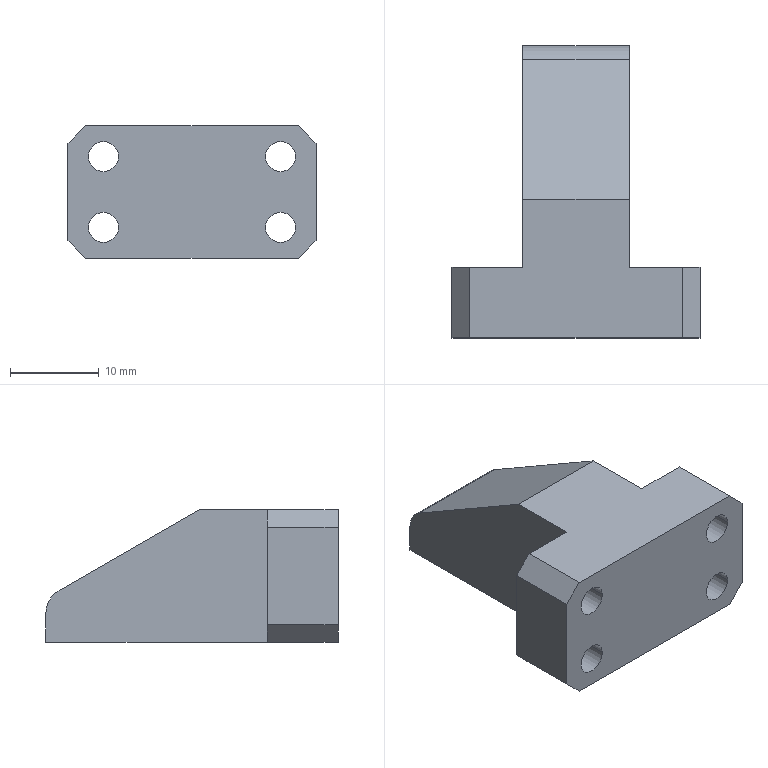Component | SolidWorks | SAWH02-03107A0MountingPlate7-5 | 1 solid | 36 faces | box 28 x 33 x 15 mm | volume 6133 mm3 | plane 19 | cylinder 17 | commonest cylinder face diameters 6.5 x8 3.4 x8 6 x1 | material SKD11
STEP:
#1=COLOUR_RGB('',0.7922,0.8196,0.9333);
#2=FILL_AREA_STYLE_COLOUR('',#1);
#3=FILL_AREA_STYLE('',(#2));
#4=SURFACE_STYLE_FILL_AREA(#3);
#5=SURFACE_SIDE_STYLE('',(#4));
#6=SURFACE_STYLE_USAGE(.BOTH.,#5);
#7=PRESENTATION_STYLE_ASSIGNMENT((#6));
#8=CARTESIAN_POINT('',(0.5614,0.1462,-4.5));
#9=VERTEX_POINT('',#8);
#10=CARTESIAN_POINT('',(0.8173,0.1462,-4.5));
#11=VERTEX_POINT('',#10);
#12=CARTESIAN_POINT('',(0.6894,0.1462,-4.5));
#13=DIRECTION('',(0.,1.,-0.));
#14=DIRECTION('',(1.,-0.,0.));
#15=AXIS2_PLACEMENT_3D('',#12,#13,#14);
#16=CIRCLE('',#15,0.128);
#17=EDGE_CURVE('',#9,#11,#16,.T.);
#18=ORIENTED_EDGE('',*,*,#17,.F.);
#19=CARTESIAN_POINT('',(0.5614,0.28,-4.5));
#20=VERTEX_POINT('',#19);
#21=CARTESIAN_POINT('',(0.5614,0.28,-4.5));
#22=DIRECTION('',(0.,1.,-0.));
#23=VECTOR('',#22,39.37);
#24=LINE('',#21,#23);
#25=EDGE_CURVE('',#9,#20,#24,.T.);
#26=ORIENTED_EDGE('',*,*,#25,.T.);
#27=CARTESIAN_POINT('',(0.8173,0.28,-4.5));
#28=VERTEX_POINT('',#27);
#29=CARTESIAN_POINT('',(0.6894,0.28,-4.5));
#30=DIRECTION('',(0.,1.,-0.));
#31=DIRECTION('',(1.,-0.,0.));
#32=AXIS2_PLACEMENT_3D('',#29,#30,#31);
#33=CIRCLE('',#32,0.128);
#34=EDGE_CURVE('',#20,#28,#33,.T.);
#35=ORIENTED_EDGE('',*,*,#34,.T.);
#36=CARTESIAN_POINT('',(0.8173,0.28,-4.5));
#37=DIRECTION('',(0.,1.,-0.));
#38=VECTOR('',#37,39.37);
#39=LINE('',#36,#38);
#40=EDGE_CURVE('',#11,#28,#39,.T.);
#41=ORIENTED_EDGE('',*,*,#40,.F.);
#42=EDGE_LOOP('',(#18,#26,#35,#41));
#43=FACE_OUTER_BOUND('',#42,.T.);
#44=CARTESIAN_POINT('',(0.6894,0.28,-4.5));
#45=DIRECTION('',(0.,1.,-0.));
#46=DIRECTION('',(1.,-0.,0.));
#47=AXIS2_PLACEMENT_3D('',#44,#45,#46);
#48=CYLINDRICAL_SURFACE('',#47,0.128);
#49=ADVANCED_FACE('',(#43),#48,.F.);
#50=CARTESIAN_POINT('',(0.6224,-0.03495,-4.5));
#51=VERTEX_POINT('',#50);
#52=CARTESIAN_POINT('',(0.7563,-0.03495,-4.5));
#53=VERTEX_POINT('',#52);
#54=CARTESIAN_POINT('',(0.6894,-0.03495,-4.5));
#55=DIRECTION('',(0.,1.,-0.));
#56=DIRECTION('',(1.,-0.,0.));
#57=AXIS2_PLACEMENT_3D('',#54,#55,#56);
#58=CIRCLE('',#57,0.06693);
#59=EDGE_CURVE('',#51,#53,#58,.T.);
#60=ORIENTED_EDGE('',*,*,#59,.F.);
#61=CARTESIAN_POINT('',(0.6224,0.1462,-4.5));
#62=VERTEX_POINT('',#61);
#63=CARTESIAN_POINT('',(0.6224,0.28,-4.5));
#64=DIRECTION('',(0.,1.,-0.));
#65=VECTOR('',#64,39.37);
#66=LINE('',#63,#65);
#67=EDGE_CURVE('',#51,#62,#66,.T.);
#68=ORIENTED_EDGE('',*,*,#67,.T.);
#69=CARTESIAN_POINT('',(0.7563,0.1462,-4.5));
#70=VERTEX_POINT('',#69);
#71=CARTESIAN_POINT('',(0.6894,0.1462,-4.5));
#72=DIRECTION('',(0.,1.,-0.));
#73=DIRECTION('',(1.,-0.,0.));
#74=AXIS2_PLACEMENT_3D('',#71,#72,#73);
#75=CIRCLE('',#74,0.06693);
#76=EDGE_CURVE('',#62,#70,#75,.T.);
#77=ORIENTED_EDGE('',*,*,#76,.T.);
#78=CARTESIAN_POINT('',(0.7563,0.28,-4.5));
#79=DIRECTION('',(0.,1.,-0.));
#80=VECTOR('',#79,39.37);
#81=LINE('',#78,#80);
#82=EDGE_CURVE('',#53,#70,#81,.T.);
#83=ORIENTED_EDGE('',*,*,#82,.F.);
#84=EDGE_LOOP('',(#60,#68,#77,#83));
#85=FACE_OUTER_BOUND('',#84,.T.);
#86=CARTESIAN_POINT('',(0.6894,0.28,-4.5));
#87=DIRECTION('',(0.,1.,-0.));
#88=DIRECTION('',(1.,0.,0.));
#89=AXIS2_PLACEMENT_3D('',#86,#87,#88);
#90=CYLINDRICAL_SURFACE('',#89,0.06693);
#91=ADVANCED_FACE('',(#85),#90,.F.);
#92=CARTESIAN_POINT('',(0.5614,0.1462,-4.815));
#93=VERTEX_POINT('',#92);
#94=CARTESIAN_POINT('',(0.8173,0.1462,-4.815));
#95=VERTEX_POINT('',#94);
#96=CARTESIAN_POINT('',(0.6894,0.1462,-4.815));
#97=DIRECTION('',(0.,1.,-0.));
#98=DIRECTION('',(1.,-0.,0.));
#99=AXIS2_PLACEMENT_3D('',#96,#97,#98);
#100=CIRCLE('',#99,0.128);
#101=EDGE_CURVE('',#93,#95,#100,.T.);
#102=ORIENTED_EDGE('',*,*,#101,.F.);
#103=CARTESIAN_POINT('',(0.5614,0.28,-4.815));
#104=VERTEX_POINT('',#103);
#105=CARTESIAN_POINT('',(0.5614,0.28,-4.815));
#106=DIRECTION('',(0.,1.,-0.));
#107=VECTOR('',#106,39.37);
#108=LINE('',#105,#107);
#109=EDGE_CURVE('',#93,#104,#108,.T.);
#110=ORIENTED_EDGE('',*,*,#109,.T.);
#111=CARTESIAN_POINT('',(0.8173,0.28,-4.815));
#112=VERTEX_POINT('',#111);
#113=CARTESIAN_POINT('',(0.6894,0.28,-4.815));
#114=DIRECTION('',(0.,1.,-0.));
#115=DIRECTION('',(1.,-0.,0.));
#116=AXIS2_PLACEMENT_3D('',#113,#114,#115);
#117=CIRCLE('',#116,0.128);
#118=EDGE_CURVE('',#104,#112,#117,.T.);
#119=ORIENTED_EDGE('',*,*,#118,.T.);
#120=CARTESIAN_POINT('',(0.8173,0.28,-4.815));
#121=DIRECTION('',(0.,1.,-0.));
#122=VECTOR('',#121,39.37);
#123=LINE('',#120,#122);
#124=EDGE_CURVE('',#95,#112,#123,.T.);
#125=ORIENTED_EDGE('',*,*,#124,.F.);
#126=EDGE_LOOP('',(#102,#110,#119,#125));
#127=FACE_OUTER_BOUND('',#126,.T.);
#128=CARTESIAN_POINT('',(0.6894,0.28,-4.815));
#129=DIRECTION('',(0.,1.,-0.));
#130=DIRECTION('',(1.,-0.,0.));
#131=AXIS2_PLACEMENT_3D('',#128,#129,#130);
#132=CYLINDRICAL_SURFACE('',#131,0.128);
#133=ADVANCED_FACE('',(#127),#132,.F.);
#134=CARTESIAN_POINT('',(0.6224,-0.03495,-4.815));
#135=VERTEX_POINT('',#134);
#136=CARTESIAN_POINT('',(0.7563,-0.03495,-4.815));
#137=VERTEX_POINT('',#136);
#138=CARTESIAN_POINT('',(0.6894,-0.03495,-4.815));
#139=DIRECTION('',(0.,1.,-0.));
#140=DIRECTION('',(1.,-0.,0.));
#141=AXIS2_PLACEMENT_3D('',#138,#139,#140);
#142=CIRCLE('',#141,0.06693);
#143=EDGE_CURVE('',#135,#137,#142,.T.);
#144=ORIENTED_EDGE('',*,*,#143,.F.);
#145=CARTESIAN_POINT('',(0.6224,0.1462,-4.815));
#146=VERTEX_POINT('',#145);
#147=CARTESIAN_POINT('',(0.6224,0.28,-4.815));
#148=DIRECTION('',(0.,1.,-0.));
#149=VECTOR('',#148,39.37);
#150=LINE('',#147,#149);
#151=EDGE_CURVE('',#135,#146,#150,.T.);
#152=ORIENTED_EDGE('',*,*,#151,.T.);
#153=CARTESIAN_POINT('',(0.7563,0.1462,-4.815));
#154=VERTEX_POINT('',#153);
#155=CARTESIAN_POINT('',(0.6894,0.1462,-4.815));
#156=DIRECTION('',(0.,1.,-0.));
#157=DIRECTION('',(1.,-0.,0.));
#158=AXIS2_PLACEMENT_3D('',#155,#156,#157);
#159=CIRCLE('',#158,0.06693);
#160=EDGE_CURVE('',#146,#154,#159,.T.);
#161=ORIENTED_EDGE('',*,*,#160,.T.);
#162=CARTESIAN_POINT('',(0.7563,0.28,-4.815));
#163=DIRECTION('',(0.,1.,-0.));
#164=VECTOR('',#163,39.37);
#165=LINE('',#162,#164);
#166=EDGE_CURVE('',#137,#154,#165,.T.);
#167=ORIENTED_EDGE('',*,*,#166,.F.);
#168=EDGE_LOOP('',(#144,#152,#161,#167));
#169=FACE_OUTER_BOUND('',#168,.T.);
#170=CARTESIAN_POINT('',(0.6894,0.28,-4.815));
#171=DIRECTION('',(0.,1.,-0.));
#172=DIRECTION('',(1.,0.,0.));
#173=AXIS2_PLACEMENT_3D('',#170,#171,#172);
#174=CYLINDRICAL_SURFACE('',#173,0.06693);
#175=ADVANCED_FACE('',(#169),#174,.F.);
#176=CARTESIAN_POINT('',(1.349,0.1462,-4.5));
#177=VERTEX_POINT('',#176);
#178=CARTESIAN_POINT('',(1.605,0.1462,-4.5));
#179=VERTEX_POINT('',#178);
#180=CARTESIAN_POINT('',(1.477,0.1462,-4.5));
#181=DIRECTION('',(0.,1.,-0.));
#182=DIRECTION('',(1.,-0.,0.));
#183=AXIS2_PLACEMENT_3D('',#180,#181,#182);
#184=CIRCLE('',#183,0.128);
#185=EDGE_CURVE('',#177,#179,#184,.T.);
#186=ORIENTED_EDGE('',*,*,#185,.F.);
#187=CARTESIAN_POINT('',(1.349,0.28,-4.5));
#188=VERTEX_POINT('',#187);
#189=CARTESIAN_POINT('',(1.349,0.28,-4.5));
#190=DIRECTION('',(0.,1.,-0.));
#191=VECTOR('',#190,39.37);
#192=LINE('',#189,#191);
#193=EDGE_CURVE('',#177,#188,#192,.T.);
#194=ORIENTED_EDGE('',*,*,#193,.T.);
#195=CARTESIAN_POINT('',(1.605,0.28,-4.5));
#196=VERTEX_POINT('',#195);
#197=CARTESIAN_POINT('',(1.477,0.28,-4.5));
#198=DIRECTION('',(0.,1.,-0.));
#199=DIRECTION('',(1.,-0.,0.));
#200=AXIS2_PLACEMENT_3D('',#197,#198,#199);
#201=CIRCLE('',#200,0.128);
#202=EDGE_CURVE('',#188,#196,#201,.T.);
#203=ORIENTED_EDGE('',*,*,#202,.T.);
#204=CARTESIAN_POINT('',(1.605,0.28,-4.5));
#205=DIRECTION('',(0.,1.,-0.));
#206=VECTOR('',#205,39.37);
#207=LINE('',#204,#206);
#208=EDGE_CURVE('',#179,#196,#207,.T.);
#209=ORIENTED_EDGE('',*,*,#208,.F.);
#210=EDGE_LOOP('',(#186,#194,#203,#209));
#211=FACE_OUTER_BOUND('',#210,.T.);
#212=CARTESIAN_POINT('',(1.477,0.28,-4.5));
#213=DIRECTION('',(0.,1.,-0.));
#214=DIRECTION('',(1.,-0.,0.));
#215=AXIS2_PLACEMENT_3D('',#212,#213,#214);
#216=CYLINDRICAL_SURFACE('',#215,0.128);
#217=ADVANCED_FACE('',(#211),#216,.F.);
#218=CARTESIAN_POINT('',(1.41,-0.03495,-4.5));
#219=VERTEX_POINT('',#218);
#220=CARTESIAN_POINT('',(1.544,-0.03495,-4.5));
#221=VERTEX_POINT('',#220);
#222=CARTESIAN_POINT('',(1.477,-0.03495,-4.5));
#223=DIRECTION('',(0.,1.,-0.));
#224=DIRECTION('',(1.,-0.,0.));
#225=AXIS2_PLACEMENT_3D('',#222,#223,#224);
#226=CIRCLE('',#225,0.06693);
#227=EDGE_CURVE('',#219,#221,#226,.T.);
#228=ORIENTED_EDGE('',*,*,#227,.F.);
#229=CARTESIAN_POINT('',(1.41,0.1462,-4.5));
#230=VERTEX_POINT('',#229);
#231=CARTESIAN_POINT('',(1.41,0.28,-4.5));
#232=DIRECTION('',(0.,1.,-0.));
#233=VECTOR('',#232,39.37);
#234=LINE('',#231,#233);
#235=EDGE_CURVE('',#219,#230,#234,.T.);
#236=ORIENTED_EDGE('',*,*,#235,.T.);
#237=CARTESIAN_POINT('',(1.544,0.1462,-4.5));
#238=VERTEX_POINT('',#237);
#239=CARTESIAN_POINT('',(1.477,0.1462,-4.5));
#240=DIRECTION('',(0.,1.,-0.));
#241=DIRECTION('',(1.,-0.,0.));
#242=AXIS2_PLACEMENT_3D('',#239,#240,#241);
#243=CIRCLE('',#242,0.06693);
#244=EDGE_CURVE('',#230,#238,#243,.T.);
#245=ORIENTED_EDGE('',*,*,#244,.T.);
#246=CARTESIAN_POINT('',(1.544,0.28,-4.5));
#247=DIRECTION('',(0.,1.,-0.));
#248=VECTOR('',#247,39.37);
#249=LINE('',#246,#248);
#250=EDGE_CURVE('',#221,#238,#249,.T.);
#251=ORIENTED_EDGE('',*,*,#250,.F.);
#252=EDGE_LOOP('',(#228,#236,#245,#251));
#253=FACE_OUTER_BOUND('',#252,.T.);
#254=CARTESIAN_POINT('',(1.477,0.28,-4.5));
#255=DIRECTION('',(0.,1.,-0.));
#256=DIRECTION('',(1.,0.,0.));
#257=AXIS2_PLACEMENT_3D('',#254,#255,#256);
#258=CYLINDRICAL_SURFACE('',#257,0.06693);
#259=ADVANCED_FACE('',(#253),#258,.F.);
#260=CARTESIAN_POINT('',(1.349,0.1462,-4.815));
#261=VERTEX_POINT('',#260);
#262=CARTESIAN_POINT('',(1.605,0.1462,-4.815));
#263=VERTEX_POINT('',#262);
#264=CARTESIAN_POINT('',(1.477,0.1462,-4.815));
#265=DIRECTION('',(0.,1.,-0.));
#266=DIRECTION('',(1.,-0.,0.));
#267=AXIS2_PLACEMENT_3D('',#264,#265,#266);
#268=CIRCLE('',#267,0.128);
#269=EDGE_CURVE('',#261,#263,#268,.T.);
#270=ORIENTED_EDGE('',*,*,#269,.F.);
#271=CARTESIAN_POINT('',(1.349,0.28,-4.815));
#272=VERTEX_POINT('',#271);
#273=CARTESIAN_POINT('',(1.349,0.28,-4.815));
#274=DIRECTION('',(0.,1.,-0.));
#275=VECTOR('',#274,39.37);
#276=LINE('',#273,#275);
#277=EDGE_CURVE('',#261,#272,#276,.T.);
#278=ORIENTED_EDGE('',*,*,#277,.T.);
#279=CARTESIAN_POINT('',(1.605,0.28,-4.815));
#280=VERTEX_POINT('',#279);
#281=CARTESIAN_POINT('',(1.477,0.28,-4.815));
#282=DIRECTION('',(0.,1.,-0.));
#283=DIRECTION('',(1.,-0.,0.));
#284=AXIS2_PLACEMENT_3D('',#281,#282,#283);
#285=CIRCLE('',#284,0.128);
#286=EDGE_CURVE('',#272,#280,#285,.T.);
#287=ORIENTED_EDGE('',*,*,#286,.T.);
#288=CARTESIAN_POINT('',(1.605,0.28,-4.815));
#289=DIRECTION('',(0.,1.,-0.));
#290=VECTOR('',#289,39.37);
#291=LINE('',#288,#290);
#292=EDGE_CURVE('',#263,#280,#291,.T.);
#293=ORIENTED_EDGE('',*,*,#292,.F.);
#294=EDGE_LOOP('',(#270,#278,#287,#293));
#295=FACE_OUTER_BOUND('',#294,.T.);
#296=CARTESIAN_POINT('',(1.477,0.28,-4.815));
#297=DIRECTION('',(0.,1.,-0.));
#298=DIRECTION('',(1.,-0.,0.));
#299=AXIS2_PLACEMENT_3D('',#296,#297,#298);
#300=CYLINDRICAL_SURFACE('',#299,0.128);
#301=ADVANCED_FACE('',(#295),#300,.F.);
#302=CARTESIAN_POINT('',(1.41,-0.03495,-4.815));
#303=VERTEX_POINT('',#302);
#304=CARTESIAN_POINT('',(1.544,-0.03495,-4.815));
#305=VERTEX_POINT('',#304);
#306=CARTESIAN_POINT('',(1.477,-0.03495,-4.815));
#307=DIRECTION('',(0.,1.,-0.));
#308=DIRECTION('',(1.,-0.,0.));
#309=AXIS2_PLACEMENT_3D('',#306,#307,#308);
#310=CIRCLE('',#309,0.06693);
#311=EDGE_CURVE('',#303,#305,#310,.T.);
#312=ORIENTED_EDGE('',*,*,#311,.F.);
#313=CARTESIAN_POINT('',(1.41,0.1462,-4.815));
#314=VERTEX_POINT('',#313);
#315=CARTESIAN_POINT('',(1.41,0.28,-4.815));
#316=DIRECTION('',(0.,1.,-0.));
#317=VECTOR('',#316,39.37);
#318=LINE('',#315,#317);
#319=EDGE_CURVE('',#303,#314,#318,.T.);
#320=ORIENTED_EDGE('',*,*,#319,.T.);
#321=CARTESIAN_POINT('',(1.544,0.1462,-4.815));
#322=VERTEX_POINT('',#321);
#323=CARTESIAN_POINT('',(1.477,0.1462,-4.815));
#324=DIRECTION('',(0.,1.,-0.));
#325=DIRECTION('',(1.,-0.,0.));
#326=AXIS2_PLACEMENT_3D('',#323,#324,#325);
#327=CIRCLE('',#326,0.06693);
#328=EDGE_CURVE('',#314,#322,#327,.T.);
#329=ORIENTED_EDGE('',*,*,#328,.T.);
#330=CARTESIAN_POINT('',(1.544,0.28,-4.815));
#331=DIRECTION('',(0.,1.,-0.));
#332=VECTOR('',#331,39.37);
#333=LINE('',#330,#332);
#334=EDGE_CURVE('',#305,#322,#333,.T.);
#335=ORIENTED_EDGE('',*,*,#334,.F.);
#336=EDGE_LOOP('',(#312,#320,#329,#335));
#337=FACE_OUTER_BOUND('',#336,.T.);
#338=CARTESIAN_POINT('',(1.477,0.28,-4.815));
#339=DIRECTION('',(0.,1.,-0.));
#340=DIRECTION('',(1.,0.,0.));
#341=AXIS2_PLACEMENT_3D('',#338,#339,#340);
#342=CYLINDRICAL_SURFACE('',#341,0.06693);
#343=ADVANCED_FACE('',(#337),#342,.F.);
#344=CARTESIAN_POINT('',(1.477,0.28,-4.5));
#345=DIRECTION('',(0.,1.,-0.));
#346=DIRECTION('',(1.,-0.,0.));
#347=AXIS2_PLACEMENT_3D('',#344,#345,#346);
#348=CIRCLE('',#347,0.128);
#349=EDGE_CURVE('',#196,#188,#348,.T.);
#350=ORIENTED_EDGE('',*,*,#349,.F.);
#351=ORIENTED_EDGE('',*,*,#202,.F.);
#352=EDGE_LOOP('',(#350,#351));
#353=FACE_BOUND('',#352,.T.);
#354=CARTESIAN_POINT('',(1.477,0.28,-4.815));
#355=DIRECTION('',(0.,1.,-0.));
#356=DIRECTION('',(1.,-0.,0.));
#357=AXIS2_PLACEMENT_3D('',#354,#355,#356);
#358=CIRCLE('',#357,0.128);
#359=EDGE_CURVE('',#280,#272,#358,.T.);
#360=ORIENTED_EDGE('',*,*,#359,.F.);
#361=ORIENTED_EDGE('',*,*,#286,.F.);
#362=EDGE_LOOP('',(#360,#361));
#363=FACE_BOUND('',#362,.T.);
#364=CARTESIAN_POINT('',(1.634,0.28,-4.441));
#365=VERTEX_POINT('',#364);
#366=CARTESIAN_POINT('',(1.634,0.28,-4.874));
#367=VERTEX_POINT('',#366);
#368=CARTESIAN_POINT('',(1.634,0.28,-4.362));
#369=DIRECTION('',(-0.,-0.,-1.));
#370=VECTOR('',#369,39.37);
#371=LINE('',#368,#370);
#372=EDGE_CURVE('',#365,#367,#371,.T.);
#373=ORIENTED_EDGE('',*,*,#372,.T.);
#374=CARTESIAN_POINT('',(1.556,0.28,-4.952));
#375=VERTEX_POINT('',#374);
#376=CARTESIAN_POINT('',(1.556,0.28,-4.952));
#377=DIRECTION('',(-0.7071,-0.,-0.7071));
#378=VECTOR('',#377,39.37);
#379=LINE('',#376,#378);
#380=EDGE_CURVE('',#367,#375,#379,.T.);
#381=ORIENTED_EDGE('',*,*,#380,.T.);
#382=CARTESIAN_POINT('',(1.319,0.28,-4.952));
#383=VERTEX_POINT('',#382);
#384=CARTESIAN_POINT('',(1.634,0.28,-4.952));
#385=DIRECTION('',(-1.,0.,0.));
#386=VECTOR('',#385,39.37);
#387=LINE('',#384,#386);
#388=EDGE_CURVE('',#375,#383,#387,.T.);
#389=ORIENTED_EDGE('',*,*,#388,.T.);
#390=CARTESIAN_POINT('',(1.319,0.28,-4.362));
#391=VERTEX_POINT('',#390);
#392=CARTESIAN_POINT('',(1.319,0.28,-4.952));
#393=DIRECTION('',(-0.,-0.,-1.));
#394=VECTOR('',#393,39.37);
#395=LINE('',#392,#394);
#396=EDGE_CURVE('',#391,#383,#395,.T.);
#397=ORIENTED_EDGE('',*,*,#396,.F.);
#398=CARTESIAN_POINT('',(1.556,0.28,-4.362));
#399=VERTEX_POINT('',#398);
#400=CARTESIAN_POINT('',(1.634,0.28,-4.362));
#401=DIRECTION('',(1.,-0.,-0.));
#402=VECTOR('',#401,39.37);
#403=LINE('',#400,#402);
#404=EDGE_CURVE('',#391,#399,#403,.T.);
#405=ORIENTED_EDGE('',*,*,#404,.T.);
#406=CARTESIAN_POINT('',(1.634,0.28,-4.441));
#407=DIRECTION('',(0.7071,-0.,-0.7071));
#408=VECTOR('',#407,39.37);
#409=LINE('',#406,#408);
#410=EDGE_CURVE('',#399,#365,#409,.T.);
#411=ORIENTED_EDGE('',*,*,#410,.T.);
#412=EDGE_LOOP('',(#373,#381,#389,#397,#405,#411));
#413=FACE_OUTER_BOUND('',#412,.T.);
#414=CARTESIAN_POINT('',(1.083,0.28,-4.657));
#415=DIRECTION('',(-0.,-1.,0.));
#416=DIRECTION('',(-1.,0.,0.));
#417=AXIS2_PLACEMENT_3D('',#414,#415,#416);
#418=PLANE('',#417);
#419=ADVANCED_FACE('',(#353,#363,#413),#418,.F.);
#420=CARTESIAN_POINT('',(0.6894,0.28,-4.5));
#421=DIRECTION('',(0.,1.,-0.));
#422=DIRECTION('',(1.,-0.,0.));
#423=AXIS2_PLACEMENT_3D('',#420,#421,#422);
#424=CIRCLE('',#423,0.128);
#425=EDGE_CURVE('',#28,#20,#424,.T.);
#426=ORIENTED_EDGE('',*,*,#425,.F.);
#427=ORIENTED_EDGE('',*,*,#34,.F.);
#428=EDGE_LOOP('',(#426,#427));
#429=FACE_BOUND('',#428,.T.);
#430=CARTESIAN_POINT('',(0.6894,0.28,-4.815));
#431=DIRECTION('',(0.,1.,-0.));
#432=DIRECTION('',(1.,-0.,0.));
#433=AXIS2_PLACEMENT_3D('',#430,#431,#432);
#434=CIRCLE('',#433,0.128);
#435=EDGE_CURVE('',#112,#104,#434,.T.);
#436=ORIENTED_EDGE('',*,*,#435,.F.);
#437=ORIENTED_EDGE('',*,*,#118,.F.);
#438=EDGE_LOOP('',(#436,#437));
#439=FACE_BOUND('',#438,.T.);
#440=CARTESIAN_POINT('',(0.8469,0.28,-4.952));
#441=VERTEX_POINT('',#440);
#442=CARTESIAN_POINT('',(0.6106,0.28,-4.952));
#443=VERTEX_POINT('',#442);
#444=CARTESIAN_POINT('',(1.634,0.28,-4.952));
#445=DIRECTION('',(-1.,0.,0.));
#446=VECTOR('',#445,39.37);
#447=LINE('',#444,#446);
#448=EDGE_CURVE('',#441,#443,#447,.T.);
#449=ORIENTED_EDGE('',*,*,#448,.T.);
#450=CARTESIAN_POINT('',(0.5319,0.28,-4.874));
#451=VERTEX_POINT('',#450);
#452=CARTESIAN_POINT('',(0.5319,0.28,-4.874));
#453=DIRECTION('',(-0.7071,0.,0.7071));
#454=VECTOR('',#453,39.37);
#455=LINE('',#452,#454);
#456=EDGE_CURVE('',#443,#451,#455,.T.);
#457=ORIENTED_EDGE('',*,*,#456,.T.);
#458=CARTESIAN_POINT('',(0.5319,0.28,-4.441));
#459=VERTEX_POINT('',#458);
#460=CARTESIAN_POINT('',(0.5319,0.28,-4.362));
#461=DIRECTION('',(0.,0.,1.));
#462=VECTOR('',#461,39.37);
#463=LINE('',#460,#462);
#464=EDGE_CURVE('',#451,#459,#463,.T.);
#465=ORIENTED_EDGE('',*,*,#464,.T.);
#466=CARTESIAN_POINT('',(0.6106,0.28,-4.362));
#467=VERTEX_POINT('',#466);
#468=CARTESIAN_POINT('',(0.6106,0.28,-4.362));
#469=DIRECTION('',(0.7071,0.,0.7071));
#470=VECTOR('',#469,39.37);
#471=LINE('',#468,#470);
#472=EDGE_CURVE('',#459,#467,#471,.T.);
#473=ORIENTED_EDGE('',*,*,#472,.T.);
#474=CARTESIAN_POINT('',(0.8469,0.28,-4.362));
#475=VERTEX_POINT('',#474);
#476=CARTESIAN_POINT('',(1.634,0.28,-4.362));
#477=DIRECTION('',(1.,-0.,-0.));
#478=VECTOR('',#477,39.37);
#479=LINE('',#476,#478);
#480=EDGE_CURVE('',#467,#475,#479,.T.);
#481=ORIENTED_EDGE('',*,*,#480,.T.);
#482=CARTESIAN_POINT('',(0.8469,0.28,-4.952));
#483=DIRECTION('',(-0.,0.,1.));
#484=VECTOR('',#483,39.37);
#485=LINE('',#482,#484);
#486=EDGE_CURVE('',#441,#475,#485,.T.);
#487=ORIENTED_EDGE('',*,*,#486,.F.);
#488=EDGE_LOOP('',(#449,#457,#465,#473,#481,#487));
#489=FACE_OUTER_BOUND('',#488,.T.);
#490=CARTESIAN_POINT('',(1.083,0.28,-4.657));
#491=DIRECTION('',(-0.,-1.,0.));
#492=DIRECTION('',(-1.,0.,0.));
#493=AXIS2_PLACEMENT_3D('',#490,#491,#492);
#494=PLANE('',#493);
#495=ADVANCED_FACE('',(#429,#439,#489),#494,.F.);
#496=ORIENTED_EDGE('',*,*,#388,.F.);
#497=CARTESIAN_POINT('',(1.556,-0.03495,-4.952));
#498=VERTEX_POINT('',#497);
#499=CARTESIAN_POINT('',(1.556,0.28,-4.952));
#500=DIRECTION('',(-0.,-1.,0.));
#501=VECTOR('',#500,39.37);
#502=LINE('',#499,#501);
#503=EDGE_CURVE('',#375,#498,#502,.T.);
#504=ORIENTED_EDGE('',*,*,#503,.T.);
#505=CARTESIAN_POINT('',(0.6106,-0.03495,-4.952));
#506=VERTEX_POINT('',#505);
#507=CARTESIAN_POINT('',(1.634,-0.03495,-4.952));
#508=DIRECTION('',(-1.,0.,0.));
#509=VECTOR('',#508,39.37);
#510=LINE('',#507,#509);
#511=EDGE_CURVE('',#498,#506,#510,.T.);
#512=ORIENTED_EDGE('',*,*,#511,.T.);
#513=CARTESIAN_POINT('',(0.6106,0.28,-4.952));
#514=DIRECTION('',(0.,1.,-0.));
#515=VECTOR('',#514,39.37);
#516=LINE('',#513,#515);
#517=EDGE_CURVE('',#506,#443,#516,.T.);
#518=ORIENTED_EDGE('',*,*,#517,.T.);
#519=ORIENTED_EDGE('',*,*,#448,.F.);
#520=CARTESIAN_POINT('',(0.8469,1.264,-4.952));
#521=VERTEX_POINT('',#520);
#522=CARTESIAN_POINT('',(0.8469,1.264,-4.952));
#523=DIRECTION('',(-0.,-1.,0.));
#524=VECTOR('',#523,39.37);
#525=LINE('',#522,#524);
#526=EDGE_CURVE('',#521,#441,#525,.T.);
#527=ORIENTED_EDGE('',*,*,#526,.F.);
#528=CARTESIAN_POINT('',(1.319,1.264,-4.952));
#529=VERTEX_POINT('',#528);
#530=CARTESIAN_POINT('',(0.8469,1.264,-4.952));
#531=DIRECTION('',(-1.,0.,0.));
#532=VECTOR('',#531,39.37);
#533=LINE('',#530,#532);
#534=EDGE_CURVE('',#529,#521,#533,.T.);
#535=ORIENTED_EDGE('',*,*,#534,.F.);
#536=CARTESIAN_POINT('',(1.319,1.264,-4.952));
#537=DIRECTION('',(-0.,-1.,0.));
#538=VECTOR('',#537,39.37);
#539=LINE('',#536,#538);
#540=EDGE_CURVE('',#529,#383,#539,.T.);
#541=ORIENTED_EDGE('',*,*,#540,.T.);
#542=EDGE_LOOP('',(#496,#504,#512,#518,#519,#527,#535,#541));
#543=FACE_OUTER_BOUND('',#542,.T.);
#544=CARTESIAN_POINT('',(1.634,0.28,-4.952));
#545=DIRECTION('',(0.,0.,1.));
#546=DIRECTION('',(1.,-0.,-0.));
#547=AXIS2_PLACEMENT_3D('',#544,#545,#546);
#548=PLANE('',#547);
#549=ADVANCED_FACE('',(#543),#548,.F.);
#550=ORIENTED_EDGE('',*,*,#464,.F.);
#551=CARTESIAN_POINT('',(0.5319,-0.03495,-4.874));
#552=VERTEX_POINT('',#551);
#553=CARTESIAN_POINT('',(0.5319,0.28,-4.874));
#554=DIRECTION('',(-0.,-1.,0.));
#555=VECTOR('',#554,39.37);
#556=LINE('',#553,#555);
#557=EDGE_CURVE('',#451,#552,#556,.T.);
#558=ORIENTED_EDGE('',*,*,#557,.T.);
#559=CARTESIAN_POINT('',(0.5319,-0.03495,-4.441));
#560=VERTEX_POINT('',#559);
#561=CARTESIAN_POINT('',(0.5319,-0.03495,-4.362));
#562=DIRECTION('',(0.,0.,1.));
#563=VECTOR('',#562,39.37);
#564=LINE('',#561,#563);
#565=EDGE_CURVE('',#552,#560,#564,.T.);
#566=ORIENTED_EDGE('',*,*,#565,.T.);
#567=CARTESIAN_POINT('',(0.5319,0.28,-4.441));
#568=DIRECTION('',(0.,1.,-0.));
#569=VECTOR('',#568,39.37);
#570=LINE('',#567,#569);
#571=EDGE_CURVE('',#560,#459,#570,.T.);
#572=ORIENTED_EDGE('',*,*,#571,.T.);
#573=EDGE_LOOP('',(#550,#558,#566,#572));
#574=FACE_OUTER_BOUND('',#573,.T.);
#575=CARTESIAN_POINT('',(0.5319,0.28,-4.362));
#576=DIRECTION('',(1.,-0.,-0.));
#577=DIRECTION('',(-0.,-0.,-1.));
#578=AXIS2_PLACEMENT_3D('',#575,#576,#577);
#579=PLANE('',#578);
#580=ADVANCED_FACE('',(#574),#579,.F.);
#581=CARTESIAN_POINT('',(0.6106,-0.03495,-4.362));
#582=VERTEX_POINT('',#581);
#583=CARTESIAN_POINT('',(1.556,-0.03495,-4.362));
#584=VERTEX_POINT('',#583);
#585=CARTESIAN_POINT('',(1.634,-0.03495,-4.362));
#586=DIRECTION('',(1.,-0.,-0.));
#587=VECTOR('',#586,39.37);
#588=LINE('',#585,#587);
#589=EDGE_CURVE('',#582,#584,#588,.T.);
#590=ORIENTED_EDGE('',*,*,#589,.T.);
#591=CARTESIAN_POINT('',(1.556,0.28,-4.362));
#592=DIRECTION('',(0.,1.,-0.));
#593=VECTOR('',#592,39.37);
#594=LINE('',#591,#593);
#595=EDGE_CURVE('',#584,#399,#594,.T.);
#596=ORIENTED_EDGE('',*,*,#595,.T.);
#597=ORIENTED_EDGE('',*,*,#404,.F.);
#598=CARTESIAN_POINT('',(1.319,0.5824,-4.362));
#599=VERTEX_POINT('',#598);
#600=CARTESIAN_POINT('',(1.319,1.264,-4.362));
#601=DIRECTION('',(-0.,-1.,0.));
#602=VECTOR('',#601,39.37);
#603=LINE('',#600,#602);
#604=EDGE_CURVE('',#599,#391,#603,.T.);
#605=ORIENTED_EDGE('',*,*,#604,.F.);
#606=CARTESIAN_POINT('',(0.8469,0.5824,-4.362));
#607=VERTEX_POINT('',#606);
#608=CARTESIAN_POINT('',(1.634,0.5824,-4.362));
#609=DIRECTION('',(-1.,0.,0.));
#610=VECTOR('',#609,39.37);
#611=LINE('',#608,#610);
#612=EDGE_CURVE('',#599,#607,#611,.T.);
#613=ORIENTED_EDGE('',*,*,#612,.T.);
#614=CARTESIAN_POINT('',(0.8469,1.264,-4.362));
#615=DIRECTION('',(-0.,-1.,0.));
#616=VECTOR('',#615,39.37);
#617=LINE('',#614,#616);
#618=EDGE_CURVE('',#607,#475,#617,.T.);
#619=ORIENTED_EDGE('',*,*,#618,.T.);
#620=ORIENTED_EDGE('',*,*,#480,.F.);
#621=CARTESIAN_POINT('',(0.6106,0.28,-4.362));
#622=DIRECTION('',(-0.,-1.,0.));
#623=VECTOR('',#622,39.37);
#624=LINE('',#621,#623);
#625=EDGE_CURVE('',#467,#582,#624,.T.);
#626=ORIENTED_EDGE('',*,*,#625,.T.);
#627=EDGE_LOOP('',(#590,#596,#597,#605,#613,#619,#620,#626));
#628=FACE_OUTER_BOUND('',#627,.T.);
#629=CARTESIAN_POINT('',(1.634,0.28,-4.362));
#630=DIRECTION('',(-0.,-0.,-1.));
#631=DIRECTION('',(-1.,0.,0.));
#632=AXIS2_PLACEMENT_3D('',#629,#630,#631);
#633=PLANE('',#632);
#634=ADVANCED_FACE('',(#628),#633,.F.);
#635=CARTESIAN_POINT('',(1.634,-0.03495,-4.441));
#636=VERTEX_POINT('',#635);
#637=CARTESIAN_POINT('',(1.634,-0.03495,-4.874));
#638=VERTEX_POINT('',#637);
#639=CARTESIAN_POINT('',(1.634,-0.03495,-4.362));
#640=DIRECTION('',(-0.,-0.,-1.));
#641=VECTOR('',#640,39.37);
#642=LINE('',#639,#641);
#643=EDGE_CURVE('',#636,#638,#642,.T.);
#644=ORIENTED_EDGE('',*,*,#643,.T.);
#645=CARTESIAN_POINT('',(1.634,0.28,-4.874));
#646=DIRECTION('',(0.,1.,-0.));
#647=VECTOR('',#646,39.37);
#648=LINE('',#645,#647);
#649=EDGE_CURVE('',#638,#367,#648,.T.);
#650=ORIENTED_EDGE('',*,*,#649,.T.);
#651=ORIENTED_EDGE('',*,*,#372,.F.);
#652=CARTESIAN_POINT('',(1.634,0.28,-4.441));
#653=DIRECTION('',(-0.,-1.,0.));
#654=VECTOR('',#653,39.37);
#655=LINE('',#652,#654);
#656=EDGE_CURVE('',#365,#636,#655,.T.);
#657=ORIENTED_EDGE('',*,*,#656,.T.);
#658=EDGE_LOOP('',(#644,#650,#651,#657));
#659=FACE_OUTER_BOUND('',#658,.T.);
#660=CARTESIAN_POINT('',(1.634,0.28,-4.362));
#661=DIRECTION('',(-1.,0.,0.));
#662=DIRECTION('',(0.,0.,1.));
#663=AXIS2_PLACEMENT_3D('',#660,#661,#662);
#664=PLANE('',#663);
#665=ADVANCED_FACE('',(#659),#664,.F.);
#666=CARTESIAN_POINT('',(0.6894,-0.03495,-4.5));
#667=DIRECTION('',(0.,1.,-0.));
#668=DIRECTION('',(1.,-0.,0.));
#669=AXIS2_PLACEMENT_3D('',#666,#667,#668);
#670=CIRCLE('',#669,0.06693);
#671=EDGE_CURVE('',#53,#51,#670,.T.);
#672=ORIENTED_EDGE('',*,*,#671,.T.);
#673=ORIENTED_EDGE('',*,*,#59,.T.);
#674=EDGE_LOOP('',(#672,#673));
#675=FACE_BOUND('',#674,.T.);
#676=CARTESIAN_POINT('',(0.6894,-0.03495,-4.815));
#677=DIRECTION('',(0.,1.,-0.));
#678=DIRECTION('',(1.,-0.,0.));
#679=AXIS2_PLACEMENT_3D('',#676,#677,#678);
#680=CIRCLE('',#679,0.06693);
#681=EDGE_CURVE('',#137,#135,#680,.T.);
#682=ORIENTED_EDGE('',*,*,#681,.T.);
#683=ORIENTED_EDGE('',*,*,#143,.T.);
#684=EDGE_LOOP('',(#682,#683));
#685=FACE_BOUND('',#684,.T.);
#686=CARTESIAN_POINT('',(1.477,-0.03495,-4.5));
#687=DIRECTION('',(0.,1.,-0.));
#688=DIRECTION('',(1.,-0.,0.));
#689=AXIS2_PLACEMENT_3D('',#686,#687,#688);
#690=CIRCLE('',#689,0.06693);
#691=EDGE_CURVE('',#221,#219,#690,.T.);
#692=ORIENTED_EDGE('',*,*,#691,.T.);
#693=ORIENTED_EDGE('',*,*,#227,.T.);
#694=EDGE_LOOP('',(#692,#693));
#695=FACE_BOUND('',#694,.T.);
#696=CARTESIAN_POINT('',(1.477,-0.03495,-4.815));
#697=DIRECTION('',(0.,1.,-0.));
#698=DIRECTION('',(1.,-0.,0.));
#699=AXIS2_PLACEMENT_3D('',#696,#697,#698);
#700=CIRCLE('',#699,0.06693);
#701=EDGE_CURVE('',#305,#303,#700,.T.);
#702=ORIENTED_EDGE('',*,*,#701,.T.);
#703=ORIENTED_EDGE('',*,*,#311,.T.);
#704=EDGE_LOOP('',(#702,#703));
#705=FACE_BOUND('',#704,.T.);
#706=ORIENTED_EDGE('',*,*,#511,.F.);
#707=CARTESIAN_POINT('',(1.467,-0.03495,-5.041));
#708=DIRECTION('',(0.7071,0.,0.7071));
#709=VECTOR('',#708,39.37);
#710=LINE('',#707,#709);
#711=EDGE_CURVE('',#498,#638,#710,.T.);
#712=ORIENTED_EDGE('',*,*,#711,.T.);
#713=ORIENTED_EDGE('',*,*,#643,.F.);
#714=CARTESIAN_POINT('',(1.467,-0.03495,-4.273));
#715=DIRECTION('',(-0.7071,0.,0.7071));
#716=VECTOR('',#715,39.37);
#717=LINE('',#714,#716);
#718=EDGE_CURVE('',#636,#584,#717,.T.);
#719=ORIENTED_EDGE('',*,*,#718,.T.);
#720=ORIENTED_EDGE('',*,*,#589,.F.);
#721=CARTESIAN_POINT('',(0.6992,-0.03495,-4.273));
#722=DIRECTION('',(-0.7071,-0.,-0.7071));
#723=VECTOR('',#722,39.37);
#724=LINE('',#721,#723);
#725=EDGE_CURVE('',#582,#560,#724,.T.);
#726=ORIENTED_EDGE('',*,*,#725,.T.);
#727=ORIENTED_EDGE('',*,*,#565,.F.);
#728=CARTESIAN_POINT('',(0.6992,-0.03495,-5.041));
#729=DIRECTION('',(0.7071,-0.,-0.7071));
#730=VECTOR('',#729,39.37);
#731=LINE('',#728,#730);
#732=EDGE_CURVE('',#552,#506,#731,.T.);
#733=ORIENTED_EDGE('',*,*,#732,.T.);
#734=EDGE_LOOP('',(#706,#712,#713,#719,#720,#726,#727,#733));
#735=FACE_OUTER_BOUND('',#734,.T.);
#736=CARTESIAN_POINT('',(1.083,-0.03495,-4.657));
#737=DIRECTION('',(-0.,-1.,0.));
#738=DIRECTION('',(-1.,0.,0.));
#739=AXIS2_PLACEMENT_3D('',#736,#737,#738);
#740=PLANE('',#739);
#741=ADVANCED_FACE('',(#675,#685,#695,#705,#735),#740,.T.);
#742=CARTESIAN_POINT('',(0.8469,1.205,-4.722));
#743=VERTEX_POINT('',#742);
#744=CARTESIAN_POINT('',(0.8469,1.264,-4.756));
#745=DIRECTION('',(0.,0.866,-0.5));
#746=VECTOR('',#745,39.37);
#747=LINE('',#744,#746);
#748=EDGE_CURVE('',#607,#743,#747,.T.);
#749=ORIENTED_EDGE('',*,*,#748,.T.);
#750=CARTESIAN_POINT('',(0.8469,1.264,-4.824));
#751=VERTEX_POINT('',#750);
#752=CARTESIAN_POINT('',(0.8469,1.146,-4.824));
#753=DIRECTION('',(-1.,0.,0.));
#754=DIRECTION('',(0.,-0.,-1.));
#755=AXIS2_PLACEMENT_3D('',#752,#753,#754);
#756=CIRCLE('',#755,0.1181);
#757=EDGE_CURVE('',#743,#751,#756,.T.);
#758=ORIENTED_EDGE('',*,*,#757,.T.);
#759=CARTESIAN_POINT('',(0.8469,1.264,-4.952));
#760=DIRECTION('',(-0.,0.,1.));
#761=VECTOR('',#760,39.37);
#762=LINE('',#759,#761);
#763=EDGE_CURVE('',#521,#751,#762,.T.);
#764=ORIENTED_EDGE('',*,*,#763,.F.);
#765=ORIENTED_EDGE('',*,*,#526,.T.);
#766=ORIENTED_EDGE('',*,*,#486,.T.);
#767=ORIENTED_EDGE('',*,*,#618,.F.);
#768=EDGE_LOOP('',(#749,#758,#764,#765,#766,#767));
#769=FACE_OUTER_BOUND('',#768,.T.);
#770=CARTESIAN_POINT('',(0.8469,1.264,-4.952));
#771=DIRECTION('',(1.,-0.,0.));
#772=DIRECTION('',(0.,-0.,-1.));
#773=AXIS2_PLACEMENT_3D('',#770,#771,#772);
#774=PLANE('',#773);
#775=ADVANCED_FACE('',(#769),#774,.F.);
#776=CARTESIAN_POINT('',(1.319,1.264,-4.824));
#777=VERTEX_POINT('',#776);
#778=CARTESIAN_POINT('',(1.319,1.264,-4.952));
#779=DIRECTION('',(-0.,-0.,-1.));
#780=VECTOR('',#779,39.37);
#781=LINE('',#778,#780);
#782=EDGE_CURVE('',#777,#529,#781,.T.);
#783=ORIENTED_EDGE('',*,*,#782,.F.);
#784=CARTESIAN_POINT('',(1.319,1.205,-4.722));
#785=VERTEX_POINT('',#784);
#786=CARTESIAN_POINT('',(1.319,1.146,-4.824));
#787=DIRECTION('',(1.,-0.,-0.));
#788=DIRECTION('',(0.,-0.,1.));
#789=AXIS2_PLACEMENT_3D('',#786,#787,#788);
#790=CIRCLE('',#789,0.1181);
#791=EDGE_CURVE('',#777,#785,#790,.T.);
#792=ORIENTED_EDGE('',*,*,#791,.T.);
#793=CARTESIAN_POINT('',(1.319,1.264,-4.756));
#794=DIRECTION('',(0.,-0.866,0.5));
#795=VECTOR('',#794,39.37);
#796=LINE('',#793,#795);
#797=EDGE_CURVE('',#785,#599,#796,.T.);
#798=ORIENTED_EDGE('',*,*,#797,.T.);
#799=ORIENTED_EDGE('',*,*,#604,.T.);
#800=ORIENTED_EDGE('',*,*,#396,.T.);
#801=ORIENTED_EDGE('',*,*,#540,.F.);
#802=EDGE_LOOP('',(#783,#792,#798,#799,#800,#801));
#803=FACE_OUTER_BOUND('',#802,.T.);
#804=CARTESIAN_POINT('',(1.319,1.264,-4.952));
#805=DIRECTION('',(-1.,0.,0.));
#806=DIRECTION('',(0.,0.,1.));
#807=AXIS2_PLACEMENT_3D('',#804,#805,#806);
#808=PLANE('',#807);
#809=ADVANCED_FACE('',(#803),#808,.F.);
#810=ORIENTED_EDGE('',*,*,#763,.T.);
#811=CARTESIAN_POINT('',(1.319,1.264,-4.824));
#812=DIRECTION('',(1.,-0.,-0.));
#813=VECTOR('',#812,39.37);
#814=LINE('',#811,#813);
#815=EDGE_CURVE('',#751,#777,#814,.T.);
#816=ORIENTED_EDGE('',*,*,#815,.T.);
#817=ORIENTED_EDGE('',*,*,#782,.T.);
#818=ORIENTED_EDGE('',*,*,#534,.T.);
#819=EDGE_LOOP('',(#810,#816,#817,#818));
#820=FACE_OUTER_BOUND('',#819,.T.);
#821=CARTESIAN_POINT('',(1.083,1.264,-4.657));
#822=DIRECTION('',(-0.,-1.,0.));
#823=DIRECTION('',(-1.,0.,0.));
#824=AXIS2_PLACEMENT_3D('',#821,#822,#823);
#825=PLANE('',#824);
#826=ADVANCED_FACE('',(#820),#825,.F.);
#827=ORIENTED_EDGE('',*,*,#797,.F.);
#828=CARTESIAN_POINT('',(0.8469,1.205,-4.722));
#829=DIRECTION('',(-1.,0.,0.));
#830=VECTOR('',#829,39.37);
#831=LINE('',#828,#830);
#832=EDGE_CURVE('',#785,#743,#831,.T.);
#833=ORIENTED_EDGE('',*,*,#832,.T.);
#834=ORIENTED_EDGE('',*,*,#748,.F.);
#835=ORIENTED_EDGE('',*,*,#612,.F.);
#836=EDGE_LOOP('',(#827,#833,#834,#835));
#837=FACE_OUTER_BOUND('',#836,.T.);
#838=CARTESIAN_POINT('',(1.083,1.264,-4.756));
#839=DIRECTION('',(-0.,-0.5,-0.866));
#840=DIRECTION('',(1.,-0.,-0.));
#841=AXIS2_PLACEMENT_3D('',#838,#839,#840);
#842=PLANE('',#841);
#843=ADVANCED_FACE('',(#837),#842,.F.);
#844=ORIENTED_EDGE('',*,*,#757,.F.);
#845=ORIENTED_EDGE('',*,*,#832,.F.);
#846=ORIENTED_EDGE('',*,*,#791,.F.);
#847=ORIENTED_EDGE('',*,*,#815,.F.);
#848=EDGE_LOOP('',(#844,#845,#846,#847));
#849=FACE_OUTER_BOUND('',#848,.T.);
#850=CARTESIAN_POINT('',(1.083,1.146,-4.824));
#851=DIRECTION('',(1.,-0.,-0.));
#852=DIRECTION('',(0.,0.,-1.));
#853=AXIS2_PLACEMENT_3D('',#850,#851,#852);
#854=CYLINDRICAL_SURFACE('',#853,0.1181);
#855=ADVANCED_FACE('',(#849),#854,.T.);
#856=ORIENTED_EDGE('',*,*,#319,.F.);
#857=ORIENTED_EDGE('',*,*,#701,.F.);
#858=ORIENTED_EDGE('',*,*,#334,.T.);
#859=CARTESIAN_POINT('',(1.477,0.1462,-4.815));
#860=DIRECTION('',(0.,1.,-0.));
#861=DIRECTION('',(1.,-0.,0.));
#862=AXIS2_PLACEMENT_3D('',#859,#860,#861);
#863=CIRCLE('',#862,0.06693);
#864=EDGE_CURVE('',#322,#314,#863,.T.);
#865=ORIENTED_EDGE('',*,*,#864,.T.);
#866=EDGE_LOOP('',(#856,#857,#858,#865));
#867=FACE_OUTER_BOUND('',#866,.T.);
#868=CARTESIAN_POINT('',(1.477,0.28,-4.815));
#869=DIRECTION('',(0.,1.,-0.));
#870=DIRECTION('',(1.,0.,0.));
#871=AXIS2_PLACEMENT_3D('',#868,#869,#870);
#872=CYLINDRICAL_SURFACE('',#871,0.06693);
#873=ADVANCED_FACE('',(#867),#872,.F.);
#874=ORIENTED_EDGE('',*,*,#864,.F.);
#875=ORIENTED_EDGE('',*,*,#328,.F.);
#876=EDGE_LOOP('',(#874,#875));
#877=FACE_BOUND('',#876,.T.);
#878=CARTESIAN_POINT('',(1.477,0.1462,-4.815));
#879=DIRECTION('',(0.,1.,-0.));
#880=DIRECTION('',(1.,-0.,0.));
#881=AXIS2_PLACEMENT_3D('',#878,#879,#880);
#882=CIRCLE('',#881,0.128);
#883=EDGE_CURVE('',#263,#261,#882,.T.);
#884=ORIENTED_EDGE('',*,*,#883,.T.);
#885=ORIENTED_EDGE('',*,*,#269,.T.);
#886=EDGE_LOOP('',(#884,#885));
#887=FACE_OUTER_BOUND('',#886,.T.);
#888=CARTESIAN_POINT('',(1.477,0.1462,-4.882));
#889=DIRECTION('',(-0.,-1.,0.));
#890=DIRECTION('',(-1.,0.,0.));
#891=AXIS2_PLACEMENT_3D('',#888,#889,#890);
#892=PLANE('',#891);
#893=ADVANCED_FACE('',(#877,#887),#892,.F.);
#894=ORIENTED_EDGE('',*,*,#277,.F.);
#895=ORIENTED_EDGE('',*,*,#883,.F.);
#896=ORIENTED_EDGE('',*,*,#292,.T.);
#897=ORIENTED_EDGE('',*,*,#359,.T.);
#898=EDGE_LOOP('',(#894,#895,#896,#897));
#899=FACE_OUTER_BOUND('',#898,.T.);
#900=CARTESIAN_POINT('',(1.477,0.28,-4.815));
#901=DIRECTION('',(0.,1.,-0.));
#902=DIRECTION('',(1.,-0.,0.));
#903=AXIS2_PLACEMENT_3D('',#900,#901,#902);
#904=CYLINDRICAL_SURFACE('',#903,0.128);
#905=ADVANCED_FACE('',(#899),#904,.F.);
#906=ORIENTED_EDGE('',*,*,#235,.F.);
#907=ORIENTED_EDGE('',*,*,#691,.F.);
#908=ORIENTED_EDGE('',*,*,#250,.T.);
#909=CARTESIAN_POINT('',(1.477,0.1462,-4.5));
#910=DIRECTION('',(0.,1.,-0.));
#911=DIRECTION('',(1.,-0.,0.));
#912=AXIS2_PLACEMENT_3D('',#909,#910,#911);
#913=CIRCLE('',#912,0.06693);
#914=EDGE_CURVE('',#238,#230,#913,.T.);
#915=ORIENTED_EDGE('',*,*,#914,.T.);
#916=EDGE_LOOP('',(#906,#907,#908,#915));
#917=FACE_OUTER_BOUND('',#916,.T.);
#918=CARTESIAN_POINT('',(1.477,0.28,-4.5));
#919=DIRECTION('',(0.,1.,-0.));
#920=DIRECTION('',(1.,0.,0.));
#921=AXIS2_PLACEMENT_3D('',#918,#919,#920);
#922=CYLINDRICAL_SURFACE('',#921,0.06693);
#923=ADVANCED_FACE('',(#917),#922,.F.);
#924=ORIENTED_EDGE('',*,*,#914,.F.);
#925=ORIENTED_EDGE('',*,*,#244,.F.);
#926=EDGE_LOOP('',(#924,#925));
#927=FACE_BOUND('',#926,.T.);
#928=CARTESIAN_POINT('',(1.477,0.1462,-4.5));
#929=DIRECTION('',(0.,1.,-0.));
#930=DIRECTION('',(1.,-0.,0.));
#931=AXIS2_PLACEMENT_3D('',#928,#929,#930);
#932=CIRCLE('',#931,0.128);
#933=EDGE_CURVE('',#179,#177,#932,.T.);
#934=ORIENTED_EDGE('',*,*,#933,.T.);
#935=ORIENTED_EDGE('',*,*,#185,.T.);
#936=EDGE_LOOP('',(#934,#935));
#937=FACE_OUTER_BOUND('',#936,.T.);
#938=CARTESIAN_POINT('',(1.477,0.1462,-4.567));
#939=DIRECTION('',(-0.,-1.,0.));
#940=DIRECTION('',(-1.,0.,0.));
#941=AXIS2_PLACEMENT_3D('',#938,#939,#940);
#942=PLANE('',#941);
#943=ADVANCED_FACE('',(#927,#937),#942,.F.);
#944=ORIENTED_EDGE('',*,*,#193,.F.);
#945=ORIENTED_EDGE('',*,*,#933,.F.);
#946=ORIENTED_EDGE('',*,*,#208,.T.);
#947=ORIENTED_EDGE('',*,*,#349,.T.);
#948=EDGE_LOOP('',(#944,#945,#946,#947));
#949=FACE_OUTER_BOUND('',#948,.T.);
#950=CARTESIAN_POINT('',(1.477,0.28,-4.5));
#951=DIRECTION('',(0.,1.,-0.));
#952=DIRECTION('',(1.,-0.,0.));
#953=AXIS2_PLACEMENT_3D('',#950,#951,#952);
#954=CYLINDRICAL_SURFACE('',#953,0.128);
#955=ADVANCED_FACE('',(#949),#954,.F.);
#956=ORIENTED_EDGE('',*,*,#151,.F.);
#957=ORIENTED_EDGE('',*,*,#681,.F.);
#958=ORIENTED_EDGE('',*,*,#166,.T.);
#959=CARTESIAN_POINT('',(0.6894,0.1462,-4.815));
#960=DIRECTION('',(0.,1.,-0.));
#961=DIRECTION('',(1.,-0.,0.));
#962=AXIS2_PLACEMENT_3D('',#959,#960,#961);
#963=CIRCLE('',#962,0.06693);
#964=EDGE_CURVE('',#154,#146,#963,.T.);
#965=ORIENTED_EDGE('',*,*,#964,.T.);
#966=EDGE_LOOP('',(#956,#957,#958,#965));
#967=FACE_OUTER_BOUND('',#966,.T.);
#968=CARTESIAN_POINT('',(0.6894,0.28,-4.815));
#969=DIRECTION('',(0.,1.,-0.));
#970=DIRECTION('',(1.,0.,0.));
#971=AXIS2_PLACEMENT_3D('',#968,#969,#970);
#972=CYLINDRICAL_SURFACE('',#971,0.06693);
#973=ADVANCED_FACE('',(#967),#972,.F.);
#974=ORIENTED_EDGE('',*,*,#964,.F.);
#975=ORIENTED_EDGE('',*,*,#160,.F.);
#976=EDGE_LOOP('',(#974,#975));
#977=FACE_BOUND('',#976,.T.);
#978=CARTESIAN_POINT('',(0.6894,0.1462,-4.815));
#979=DIRECTION('',(0.,1.,-0.));
#980=DIRECTION('',(1.,-0.,0.));
#981=AXIS2_PLACEMENT_3D('',#978,#979,#980);
#982=CIRCLE('',#981,0.128);
#983=EDGE_CURVE('',#95,#93,#982,.T.);
#984=ORIENTED_EDGE('',*,*,#983,.T.);
#985=ORIENTED_EDGE('',*,*,#101,.T.);
#986=EDGE_LOOP('',(#984,#985));
#987=FACE_OUTER_BOUND('',#986,.T.);
#988=CARTESIAN_POINT('',(0.6894,0.1462,-4.882));
#989=DIRECTION('',(-0.,-1.,0.));
#990=DIRECTION('',(-1.,0.,0.));
#991=AXIS2_PLACEMENT_3D('',#988,#989,#990);
#992=PLANE('',#991);
#993=ADVANCED_FACE('',(#977,#987),#992,.F.);
#994=ORIENTED_EDGE('',*,*,#109,.F.);
#995=ORIENTED_EDGE('',*,*,#983,.F.);
#996=ORIENTED_EDGE('',*,*,#124,.T.);
#997=ORIENTED_EDGE('',*,*,#435,.T.);
#998=EDGE_LOOP('',(#994,#995,#996,#997));
#999=FACE_OUTER_BOUND('',#998,.T.);
#1000=CARTESIAN_POINT('',(0.6894,0.28,-4.815));
#1001=DIRECTION('',(0.,1.,-0.));
#1002=DIRECTION('',(1.,-0.,0.));
#1003=AXIS2_PLACEMENT_3D('',#1000,#1001,#1002);
#1004=CYLINDRICAL_SURFACE('',#1003,0.128);
#1005=ADVANCED_FACE('',(#999),#1004,.F.);
#1006=ORIENTED_EDGE('',*,*,#67,.F.);
#1007=ORIENTED_EDGE('',*,*,#671,.F.);
#1008=ORIENTED_EDGE('',*,*,#82,.T.);
#1009=CARTESIAN_POINT('',(0.6894,0.1462,-4.5));
#1010=DIRECTION('',(0.,1.,-0.));
#1011=DIRECTION('',(1.,-0.,0.));
#1012=AXIS2_PLACEMENT_3D('',#1009,#1010,#1011);
#1013=CIRCLE('',#1012,0.06693);
#1014=EDGE_CURVE('',#70,#62,#1013,.T.);
#1015=ORIENTED_EDGE('',*,*,#1014,.T.);
#1016=EDGE_LOOP('',(#1006,#1007,#1008,#1015));
#1017=FACE_OUTER_BOUND('',#1016,.T.);
#1018=CARTESIAN_POINT('',(0.6894,0.28,-4.5));
#1019=DIRECTION('',(0.,1.,-0.));
#1020=DIRECTION('',(1.,0.,0.));
#1021=AXIS2_PLACEMENT_3D('',#1018,#1019,#1020);
#1022=CYLINDRICAL_SURFACE('',#1021,0.06693);
#1023=ADVANCED_FACE('',(#1017),#1022,.F.);
#1024=ORIENTED_EDGE('',*,*,#1014,.F.);
#1025=ORIENTED_EDGE('',*,*,#76,.F.);
#1026=EDGE_LOOP('',(#1024,#1025));
#1027=FACE_BOUND('',#1026,.T.);
#1028=CARTESIAN_POINT('',(0.6894,0.1462,-4.5));
#1029=DIRECTION('',(0.,1.,-0.));
#1030=DIRECTION('',(1.,-0.,0.));
#1031=AXIS2_PLACEMENT_3D('',#1028,#1029,#1030);
#1032=CIRCLE('',#1031,0.128);
#1033=EDGE_CURVE('',#11,#9,#1032,.T.);
#1034=ORIENTED_EDGE('',*,*,#1033,.T.);
#1035=ORIENTED_EDGE('',*,*,#17,.T.);
#1036=EDGE_LOOP('',(#1034,#1035));
#1037=FACE_OUTER_BOUND('',#1036,.T.);
#1038=CARTESIAN_POINT('',(0.6894,0.1462,-4.567));
#1039=DIRECTION('',(-0.,-1.,0.));
#1040=DIRECTION('',(-1.,0.,0.));
#1041=AXIS2_PLACEMENT_3D('',#1038,#1039,#1040);
#1042=PLANE('',#1041);
#1043=ADVANCED_FACE('',(#1027,#1037),#1042,.F.);
#1044=ORIENTED_EDGE('',*,*,#25,.F.);
#1045=ORIENTED_EDGE('',*,*,#1033,.F.);
#1046=ORIENTED_EDGE('',*,*,#40,.T.);
#1047=ORIENTED_EDGE('',*,*,#425,.T.);
#1048=EDGE_LOOP('',(#1044,#1045,#1046,#1047));
#1049=FACE_OUTER_BOUND('',#1048,.T.);
#1050=CARTESIAN_POINT('',(0.6894,0.28,-4.5));
#1051=DIRECTION('',(0.,1.,-0.));
#1052=DIRECTION('',(1.,-0.,0.));
#1053=AXIS2_PLACEMENT_3D('',#1050,#1051,#1052);
#1054=CYLINDRICAL_SURFACE('',#1053,0.128);
#1055=ADVANCED_FACE('',(#1049),#1054,.F.);
#1056=ORIENTED_EDGE('',*,*,#380,.F.);
#1057=ORIENTED_EDGE('',*,*,#649,.F.);
#1058=ORIENTED_EDGE('',*,*,#711,.F.);
#1059=ORIENTED_EDGE('',*,*,#503,.F.);
#1060=EDGE_LOOP('',(#1056,#1057,#1058,#1059));
#1061=FACE_OUTER_BOUND('',#1060,.T.);
#1062=CARTESIAN_POINT('',(1.556,0.28,-4.952));
#1063=DIRECTION('',(-0.7071,0.,0.7071));
#1064=DIRECTION('',(-0.,-1.,0.));
#1065=AXIS2_PLACEMENT_3D('',#1062,#1063,#1064);
#1066=PLANE('',#1065);
#1067=ADVANCED_FACE('',(#1061),#1066,.F.);
#1068=ORIENTED_EDGE('',*,*,#410,.F.);
#1069=ORIENTED_EDGE('',*,*,#595,.F.);
#1070=ORIENTED_EDGE('',*,*,#718,.F.);
#1071=ORIENTED_EDGE('',*,*,#656,.F.);
#1072=EDGE_LOOP('',(#1068,#1069,#1070,#1071));
#1073=FACE_OUTER_BOUND('',#1072,.T.);
#1074=CARTESIAN_POINT('',(1.634,0.28,-4.441));
#1075=DIRECTION('',(-0.7071,-0.,-0.7071));
#1076=DIRECTION('',(-0.,-1.,0.));
#1077=AXIS2_PLACEMENT_3D('',#1074,#1075,#1076);
#1078=PLANE('',#1077);
#1079=ADVANCED_FACE('',(#1073),#1078,.F.);
#1080=ORIENTED_EDGE('',*,*,#456,.F.);
#1081=ORIENTED_EDGE('',*,*,#517,.F.);
#1082=ORIENTED_EDGE('',*,*,#732,.F.);
#1083=ORIENTED_EDGE('',*,*,#557,.F.);
#1084=EDGE_LOOP('',(#1080,#1081,#1082,#1083));
#1085=FACE_OUTER_BOUND('',#1084,.T.);
#1086=CARTESIAN_POINT('',(0.5319,0.28,-4.874));
#1087=DIRECTION('',(0.7071,0.,0.7071));
#1088=DIRECTION('',(-0.,-1.,0.));
#1089=AXIS2_PLACEMENT_3D('',#1086,#1087,#1088);
#1090=PLANE('',#1089);
#1091=ADVANCED_FACE('',(#1085),#1090,.F.);
#1092=ORIENTED_EDGE('',*,*,#472,.F.);
#1093=ORIENTED_EDGE('',*,*,#571,.F.);
#1094=ORIENTED_EDGE('',*,*,#725,.F.);
#1095=ORIENTED_EDGE('',*,*,#625,.F.);
#1096=EDGE_LOOP('',(#1092,#1093,#1094,#1095));
#1097=FACE_OUTER_BOUND('',#1096,.T.);
#1098=CARTESIAN_POINT('',(0.6106,0.28,-4.362));
#1099=DIRECTION('',(0.7071,-0.,-0.7071));
#1100=DIRECTION('',(-0.,-1.,0.));
#1101=AXIS2_PLACEMENT_3D('',#1098,#1099,#1100);
#1102=PLANE('',#1101);
#1103=ADVANCED_FACE('',(#1097),#1102,.F.);
#1104=CLOSED_SHELL('',(#49,#91,#133,#175,#217,#259,#301,#343,#419,#495,#549,#580,#634,#665,#741,#775,#809,#826,#843,#855,#873,#893,#905,#923,#943,#955,#973,#993,#1005,#1023,#1043,#1055,#1067,#1079,#1091,#1103));
#1105=MANIFOLD_SOLID_BREP('',#1104);
#1106=STYLED_ITEM('',(#7),#1105);
#1107=PRESENTATION_LAYER_ASSIGNMENT('','',(#1106));
#1108=CARTESIAN_POINT('',(0.,0.,0.));
#1109=DIRECTION('',(0.,0.,1.));
#1110=DIRECTION('',(1.,0.,0.));
#1111=AXIS2_PLACEMENT_3D('',#1108,#1109,#1110);
#1112=(LENGTH_UNIT()NAMED_UNIT(*)SI_UNIT($,.METRE.));
#1113=LENGTH_MEASURE_WITH_UNIT(LENGTH_MEASURE(0.0254),#1112);
#1114=DIMENSIONAL_EXPONENTS(1.,0.,0.,0.,0.,0.,0.);
#1115=(CONVERSION_BASED_UNIT('',#1113)LENGTH_UNIT()NAMED_UNIT(#1114));
#1116=UNCERTAINTY_MEASURE_WITH_UNIT(LENGTH_MEASURE(0.00001),#1115,'','');
#1117=(NAMED_UNIT(*)PLANE_ANGLE_UNIT()SI_UNIT($,.RADIAN.));
#1118=(NAMED_UNIT(*)SI_UNIT($,.STERADIAN.)SOLID_ANGLE_UNIT());
#1119=(GEOMETRIC_REPRESENTATION_CONTEXT(3)GLOBAL_UNCERTAINTY_ASSIGNED_CONTEXT((#1116))GLOBAL_UNIT_ASSIGNED_CONTEXT((#1115,#1117,#1118))REPRESENTATION_CONTEXT('',''));
#1120=ADVANCED_BREP_SHAPE_REPRESENTATION('',(#1105,#1111),#1119);
#1121=(LENGTH_UNIT()NAMED_UNIT(*)SI_UNIT($,.METRE.));
#1122=LENGTH_MEASURE_WITH_UNIT(LENGTH_MEASURE(0.0254),#1121);
#1123=DIMENSIONAL_EXPONENTS(1.,0.,0.,0.,0.,0.,0.);
#1124=(CONVERSION_BASED_UNIT('',#1122)LENGTH_UNIT()NAMED_UNIT(#1123));
#1125=UNCERTAINTY_MEASURE_WITH_UNIT(LENGTH_MEASURE(0.00001),#1124,'','');
#1126=(NAMED_UNIT(*)PLANE_ANGLE_UNIT()SI_UNIT($,.RADIAN.));
#1127=(NAMED_UNIT(*)SI_UNIT($,.STERADIAN.)SOLID_ANGLE_UNIT());
#1128=(GEOMETRIC_REPRESENTATION_CONTEXT(3)GLOBAL_UNCERTAINTY_ASSIGNED_CONTEXT((#1125))GLOBAL_UNIT_ASSIGNED_CONTEXT((#1124,#1126,#1127))REPRESENTATION_CONTEXT('',''));
#1129=MECHANICAL_DESIGN_GEOMETRIC_PRESENTATION_REPRESENTATION('',(#1106),#1128);